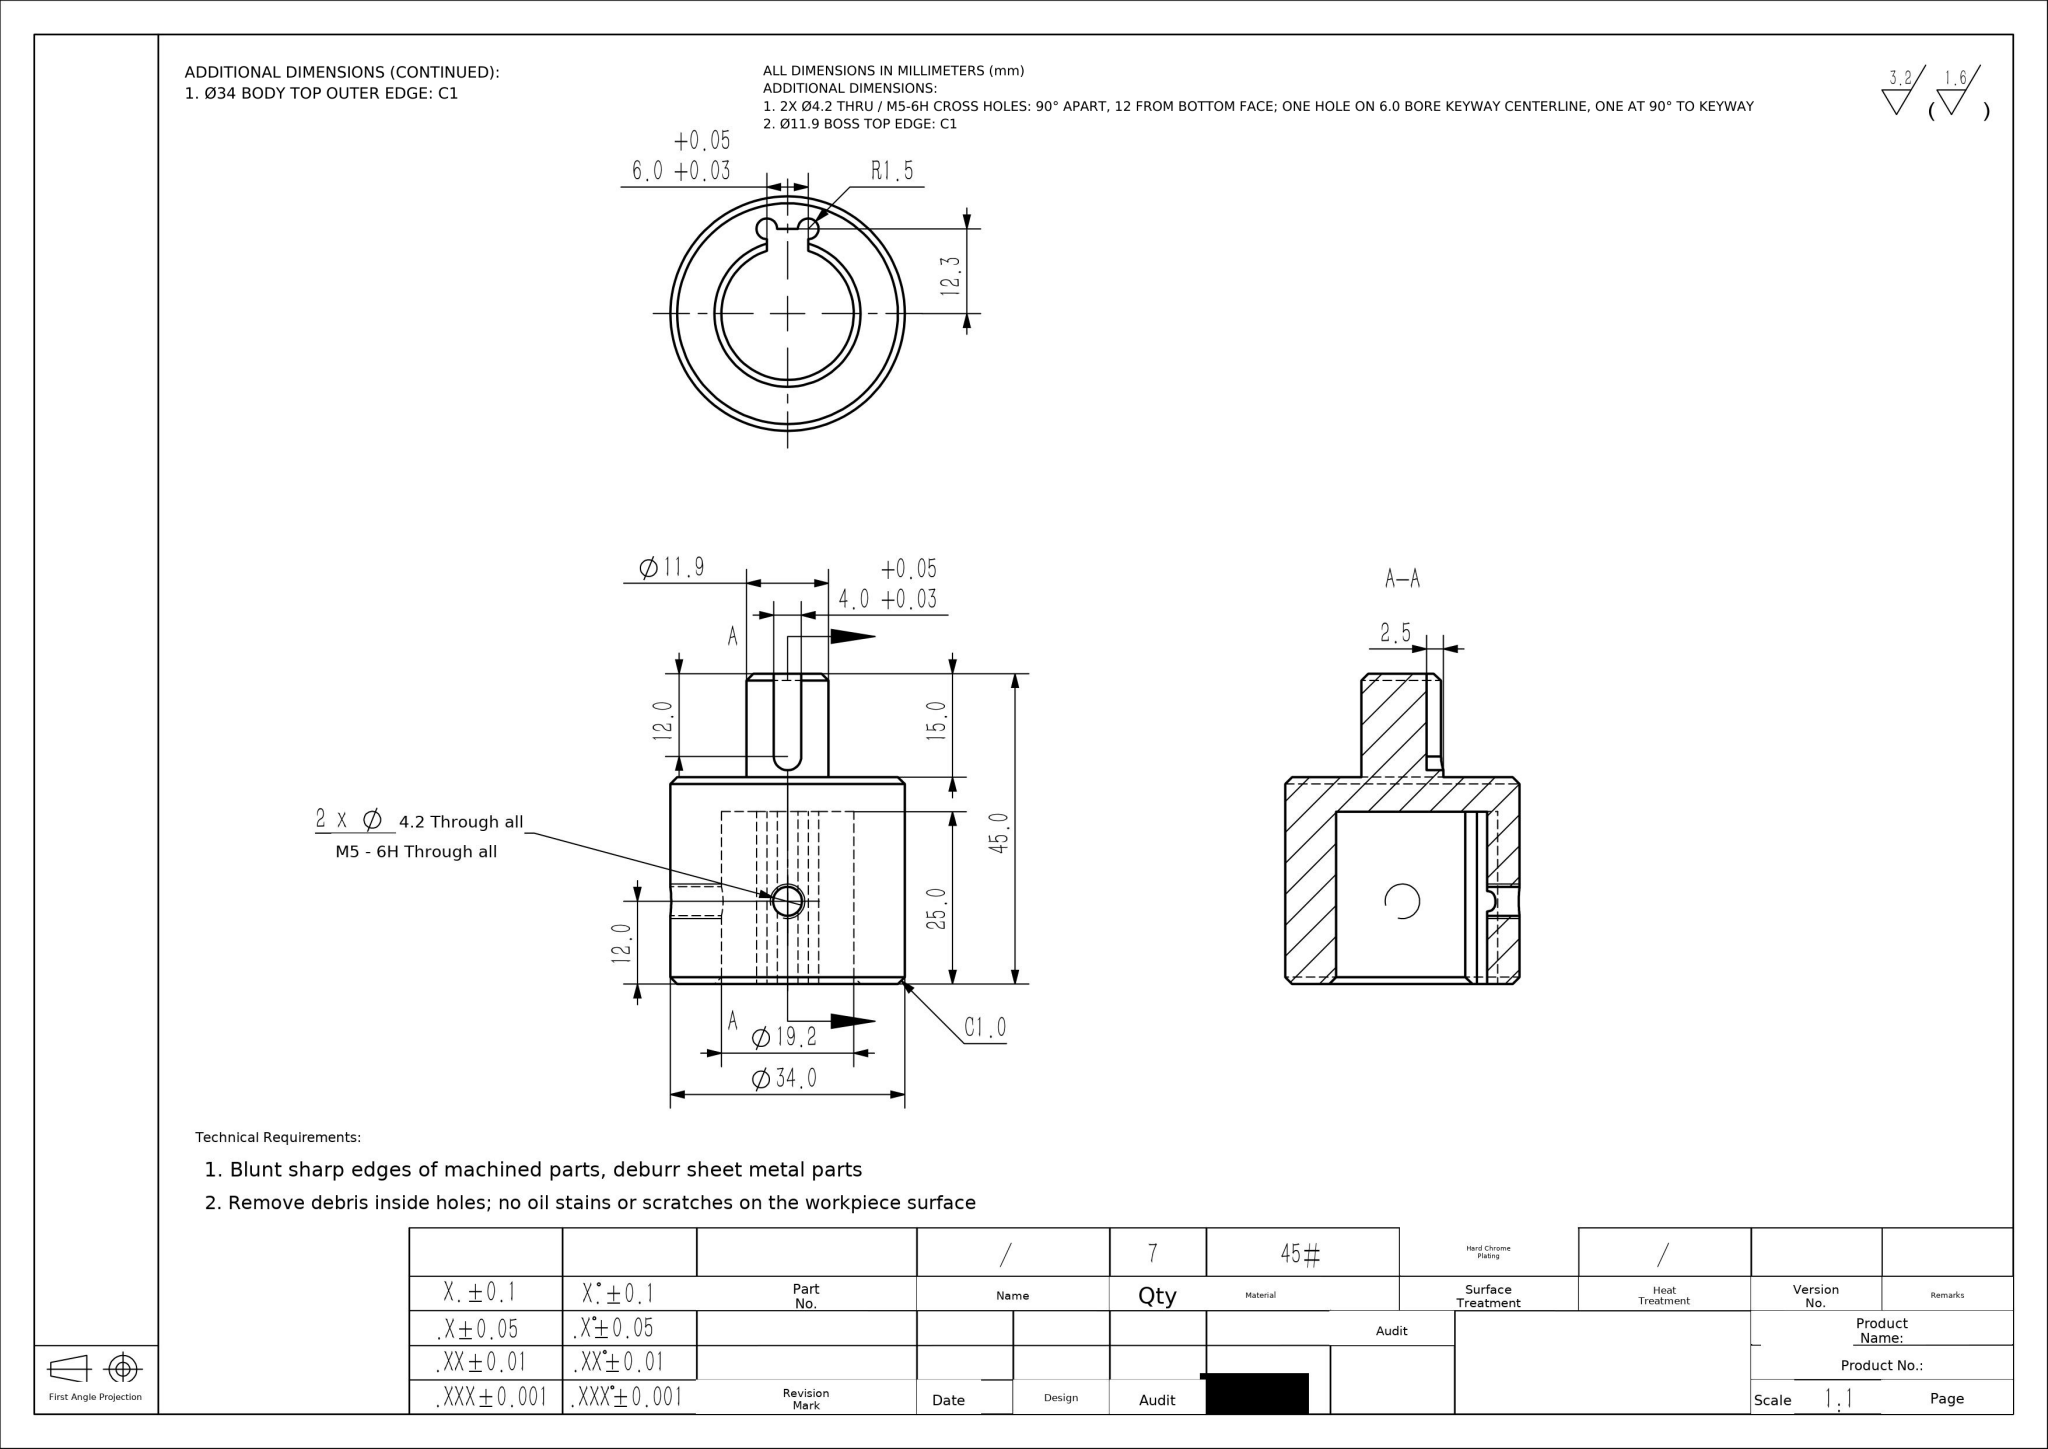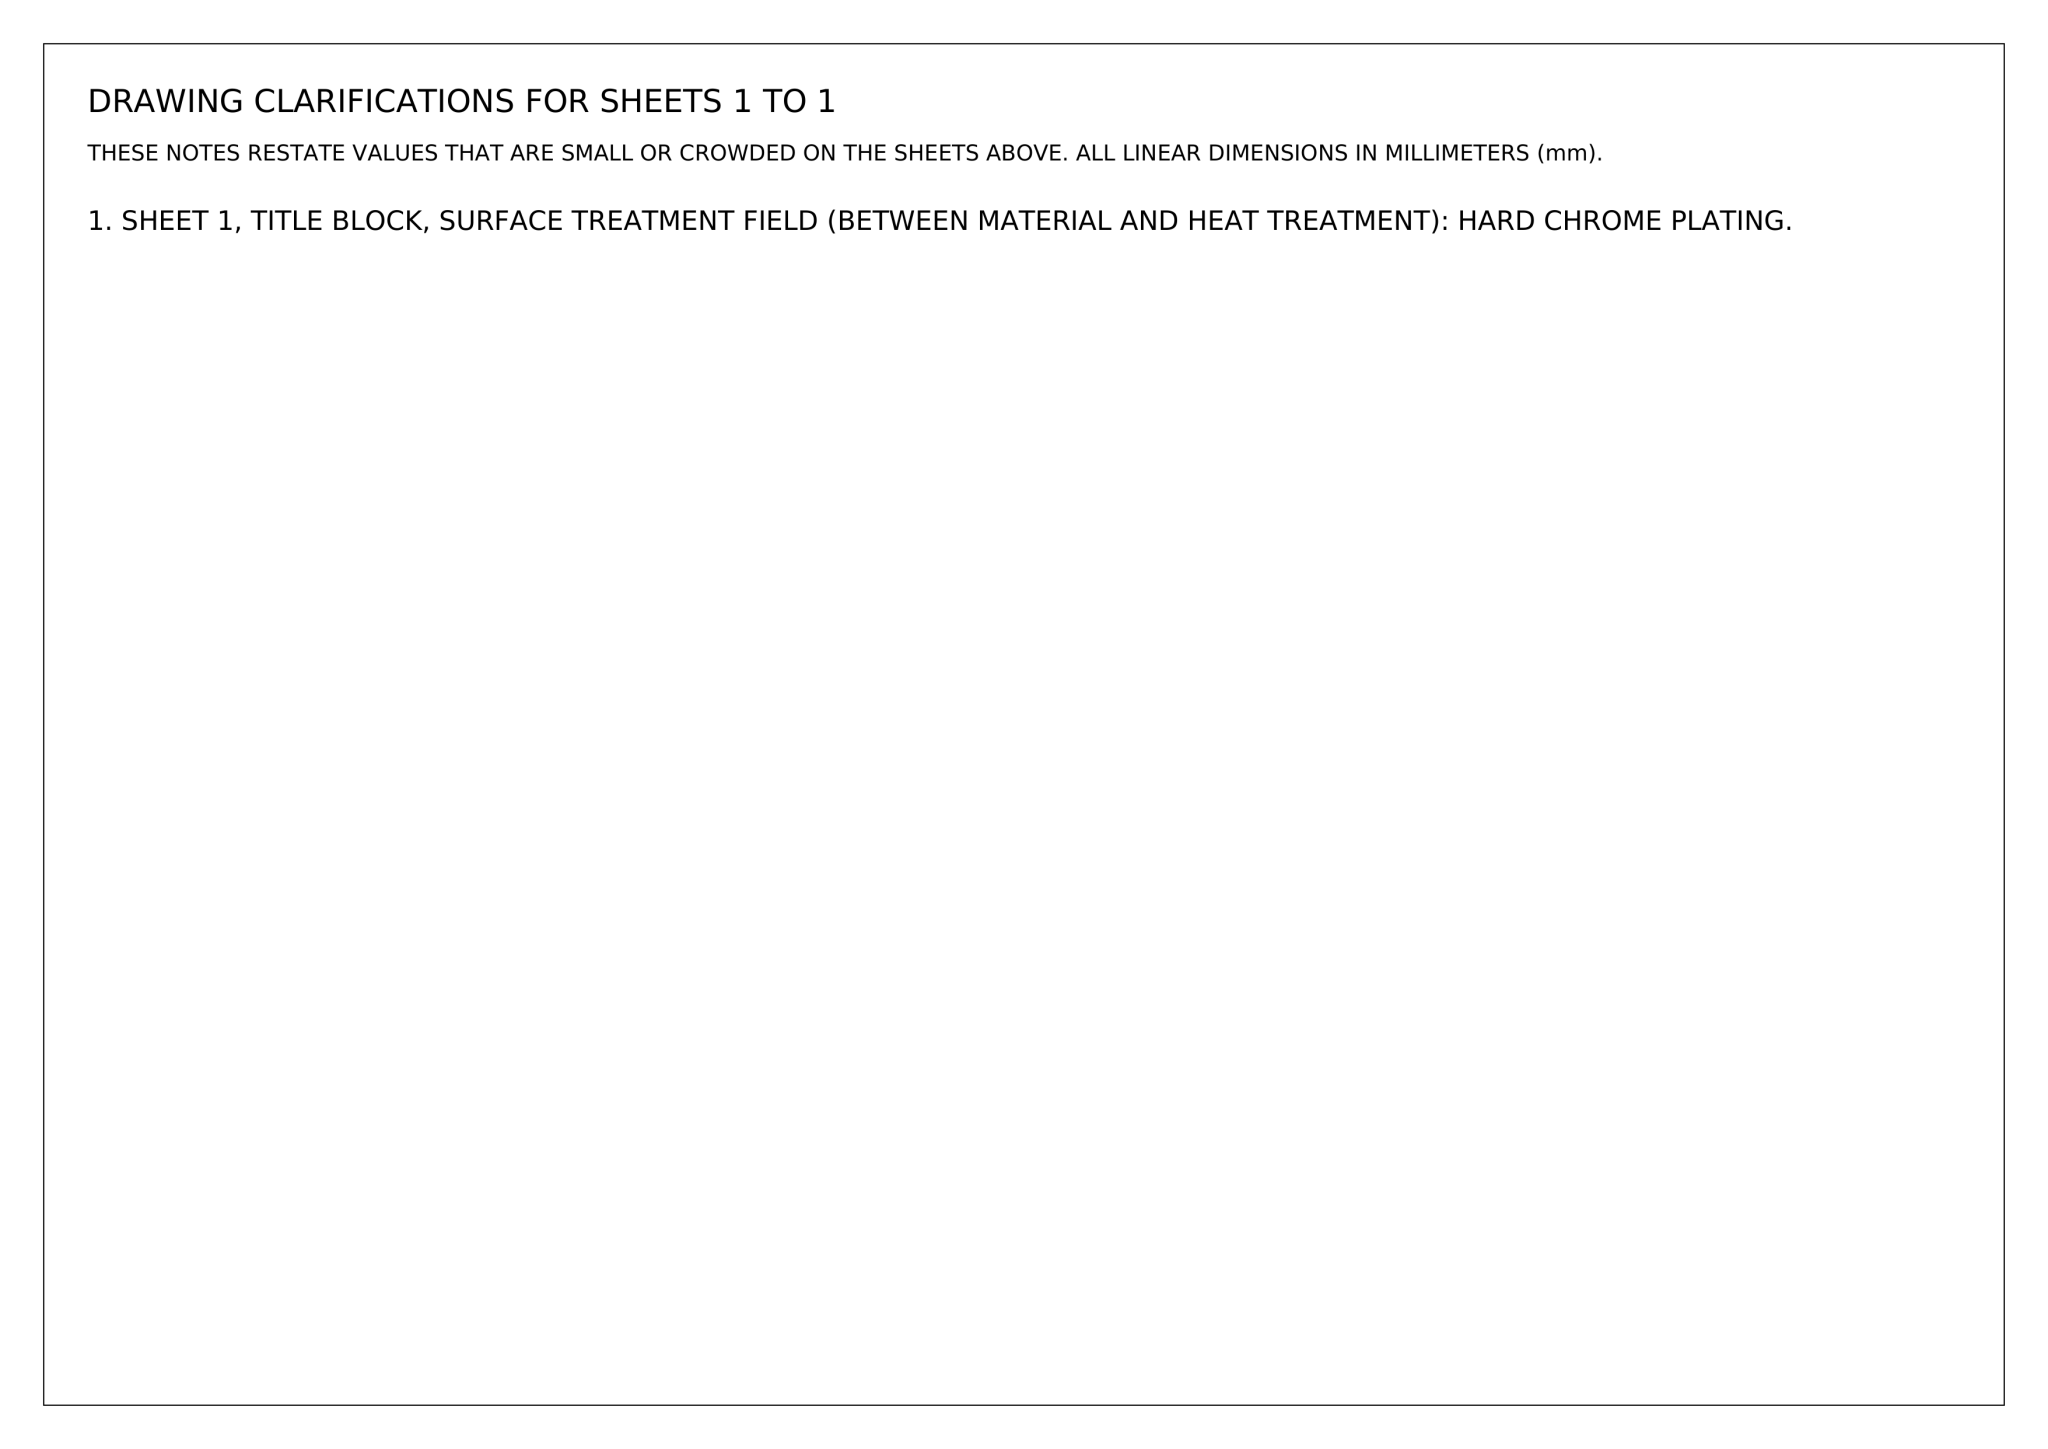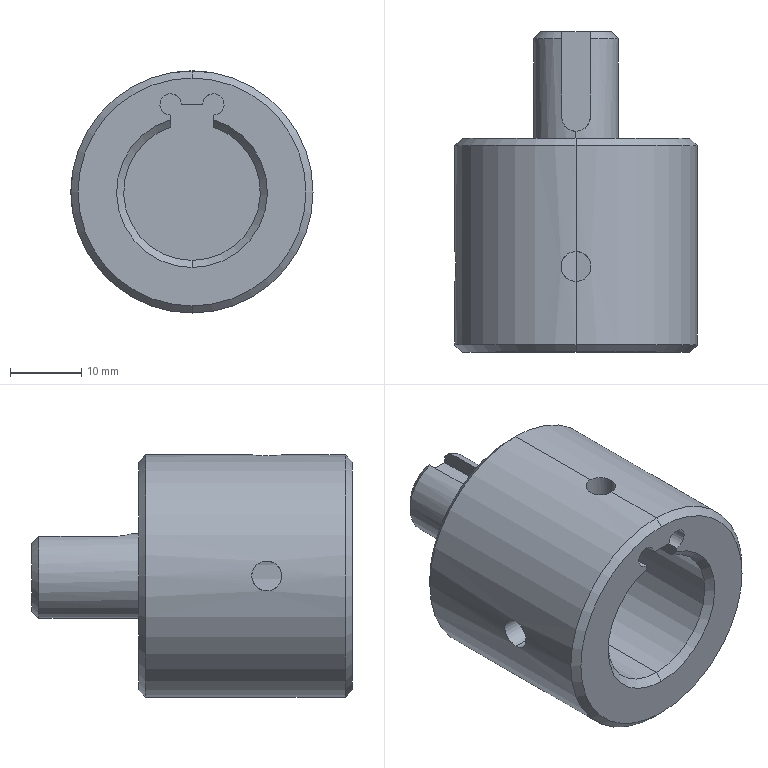Part | NX | mm | 1 solid | 32 faces | box 34 x 45 x 34 mm | volume 20533 mm3 | cylinder 13 | plane 11 | cone 8 | commonest cylinder face diameters 4.2 x4 19.2 x2 34 x2 11.9 x2 3 x2 4 x1